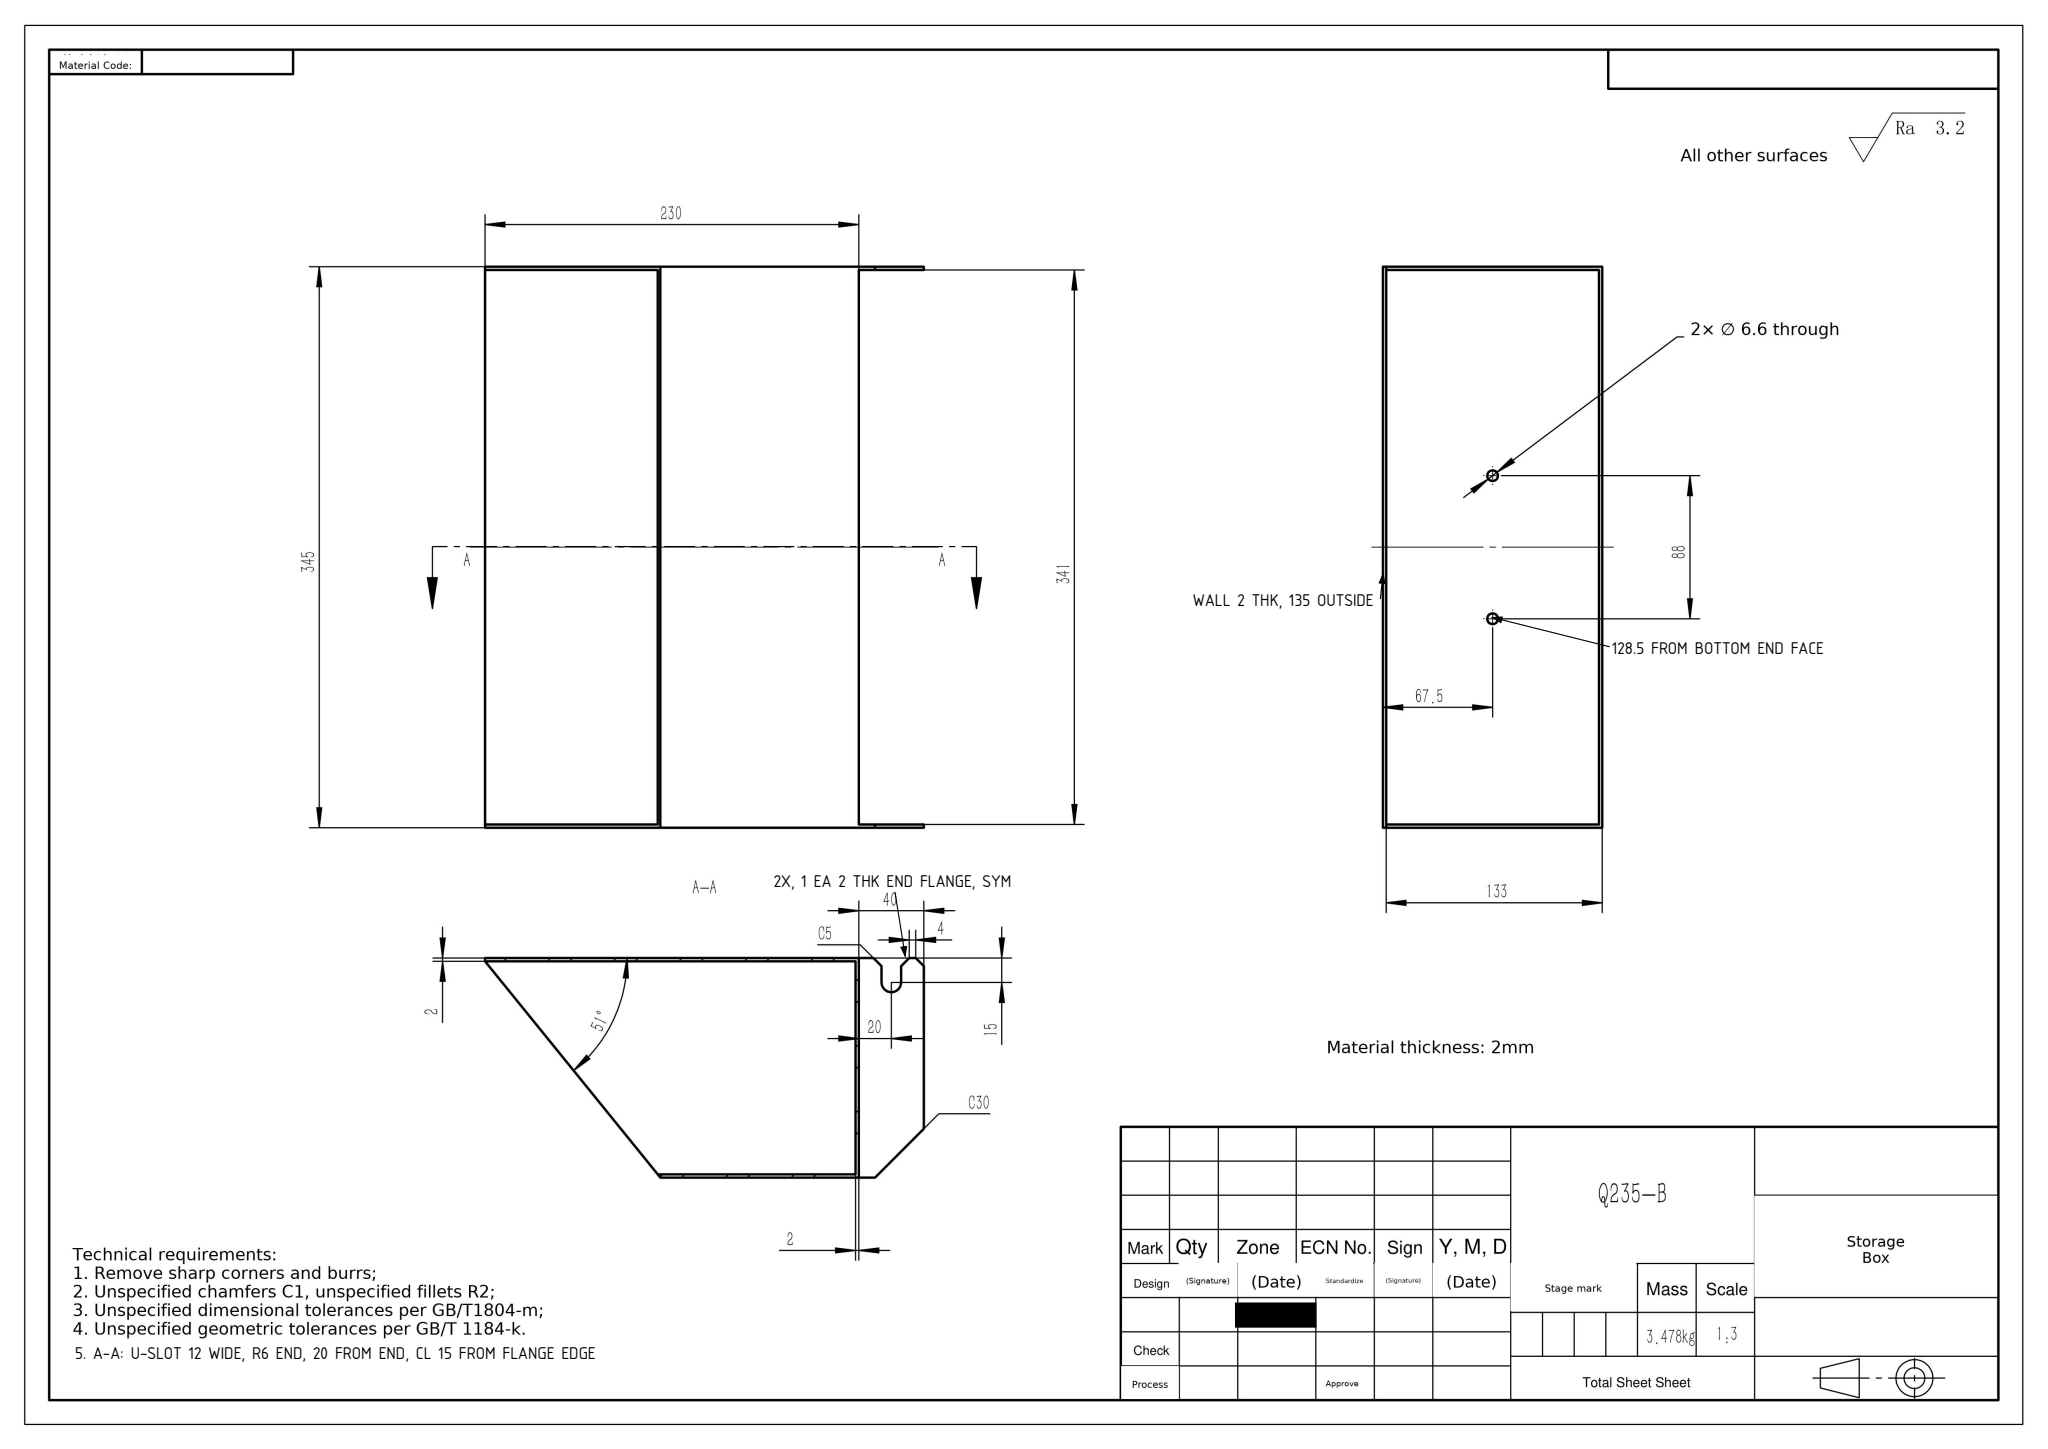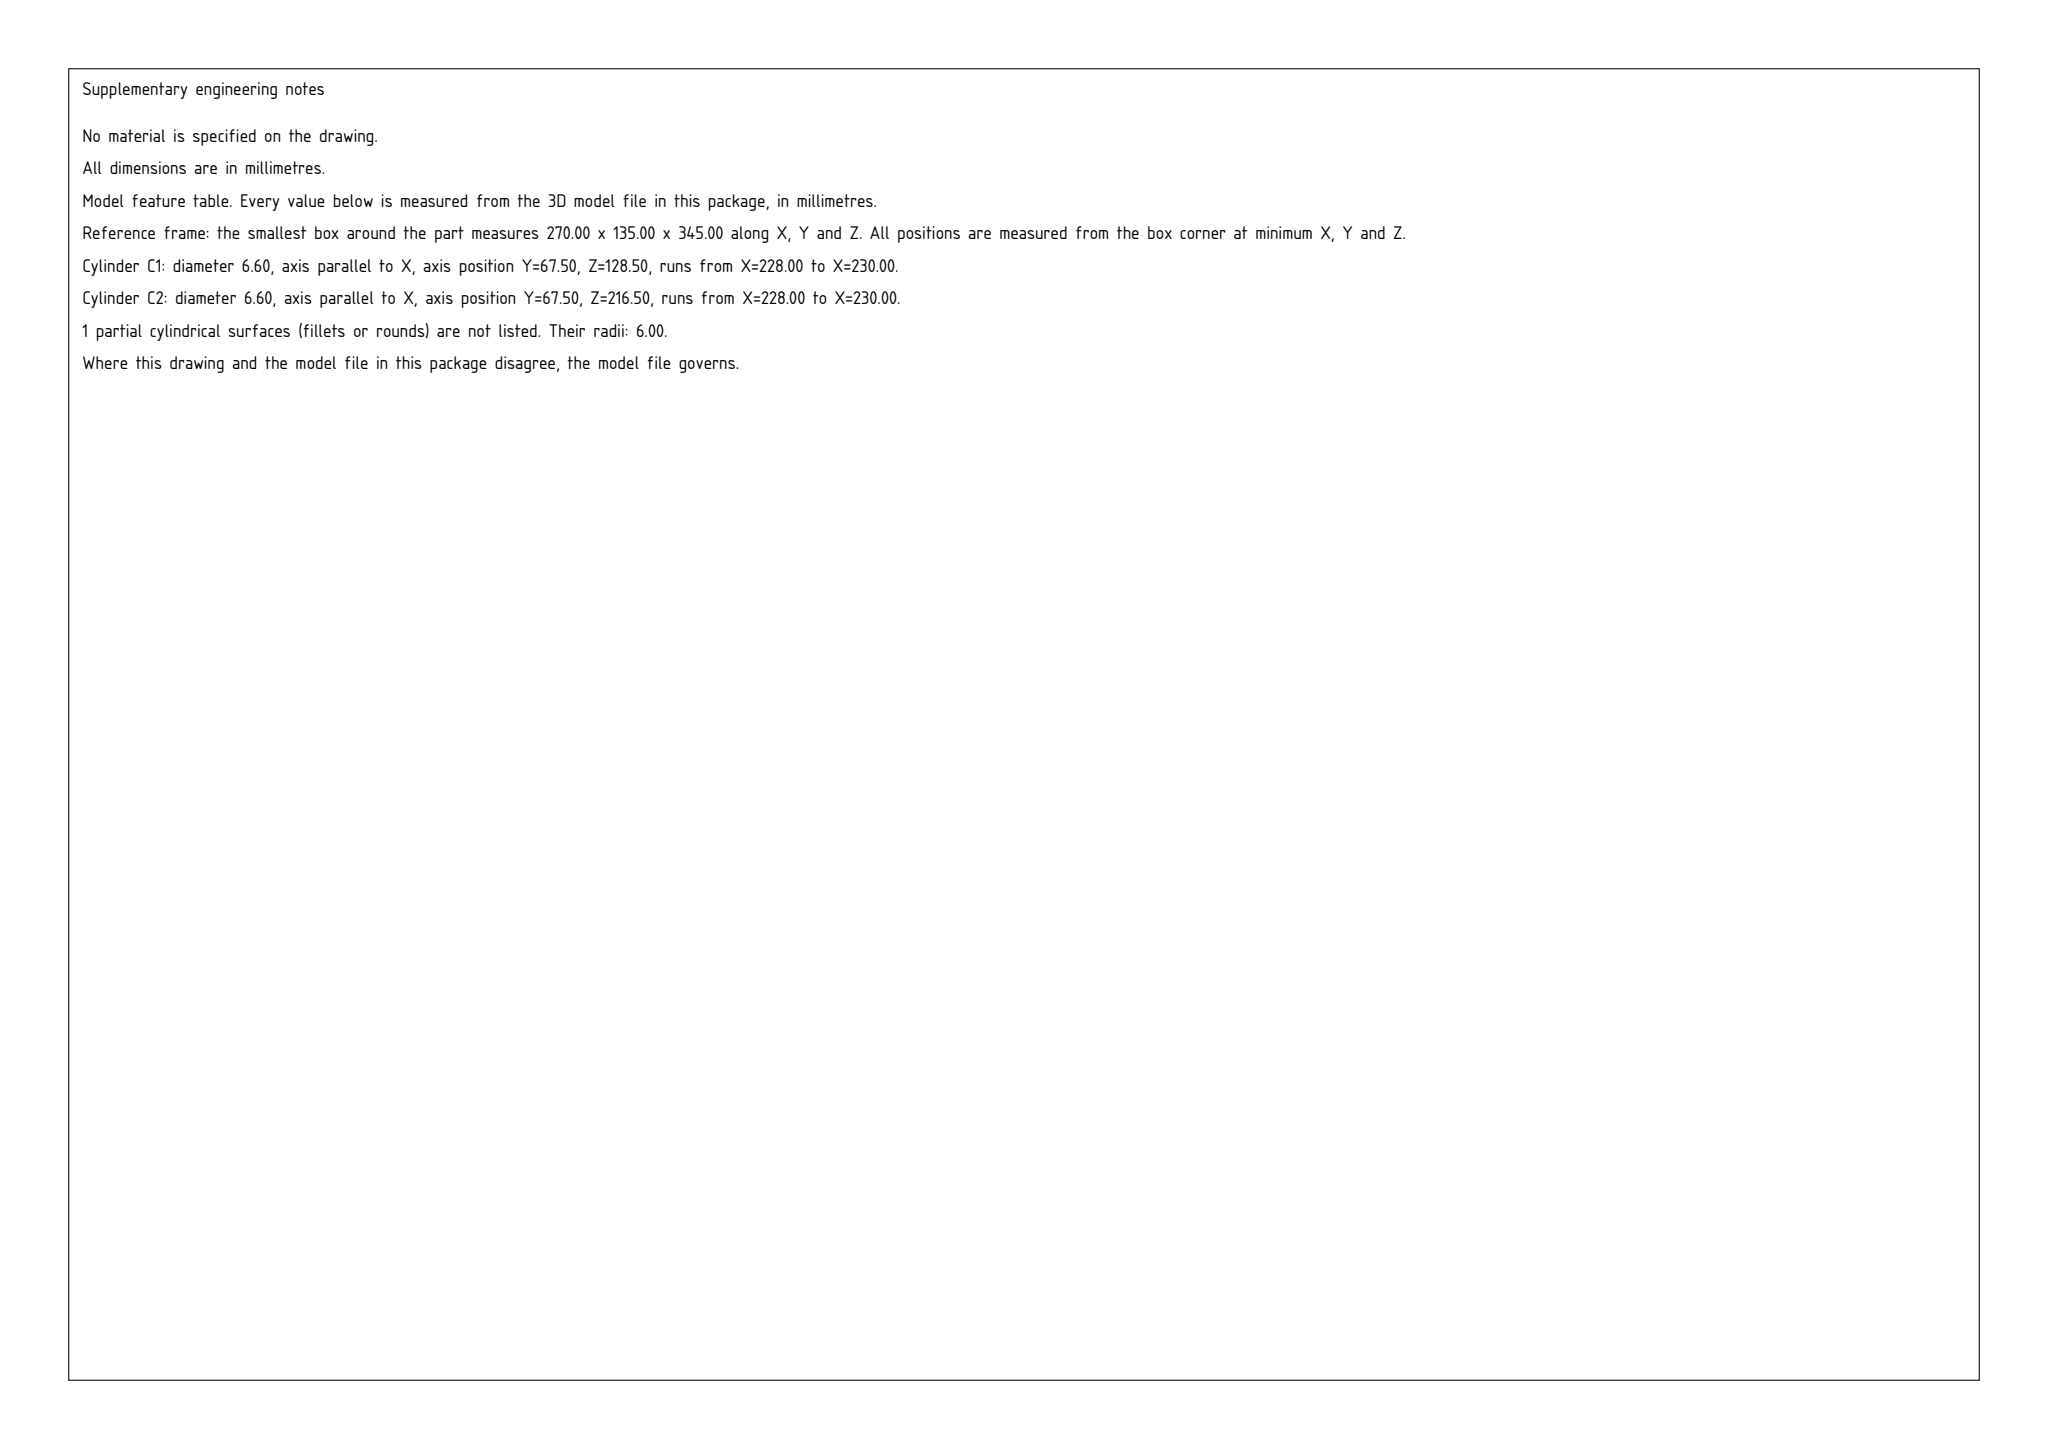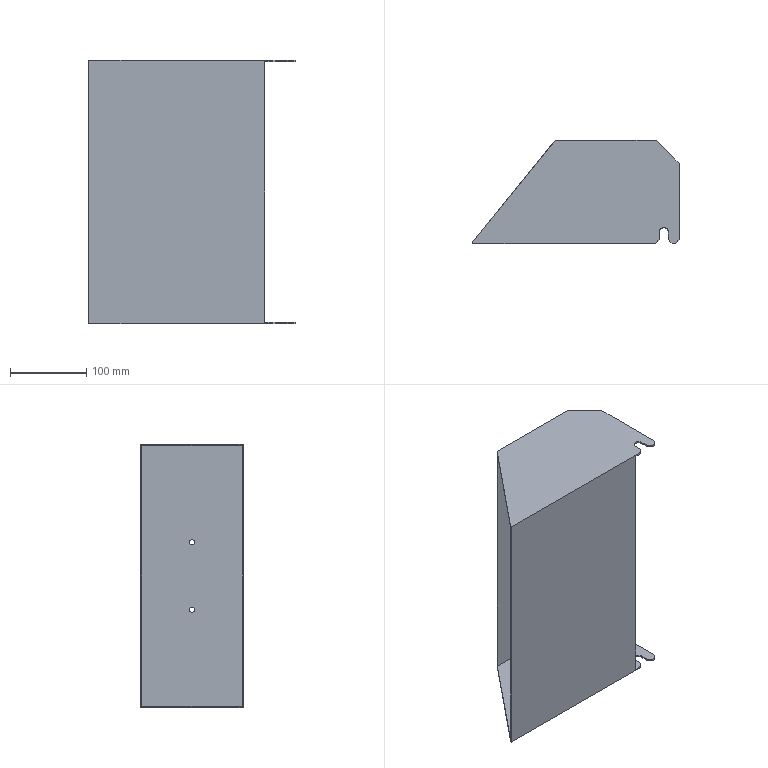Part | SolidWorks | mm | material Q235-B | 1 solid | 36 faces | box 270 x 135 x 345 mm | volume 444127 mm3 | plane 30 | cylinder 6 | commonest cylinder face diameters 6.6 x4 12 x2
Drawing notes:
A-A: U-SLOT 12 WIDE, R6 END, 20 FROM END, CL 15 FROM FLANGE EDGE | from the solid: cylinder dia 12 axis z at (x=250, y=15), len 2; bbox x=270 so 20 from end face; flange face y=0
2X U-SLOT: 1 IN EA 2 THK END FLANGE (Z 0-2 & 343-345), SYM | from the solid: [[12.0,"z",[250.0,15.0,null],2.0,2]] count=2; planes z=0,2 and z=343,345
SIDE VIEW: OVERALL WIDTH 135 OUTSIDE (133 INSIDE), 2 THK WALL | from the solid: y planes at 0, 2, 133, 135 -> bbox Y = 135, wall 2
2X Ø6.6 THRU: 128.5 FROM BOTTOM END FACE, 88 APART | from the solid: Ø6.6 x-axis cyls at z=128.5 and z=216.5; z face at 0; 345 overall